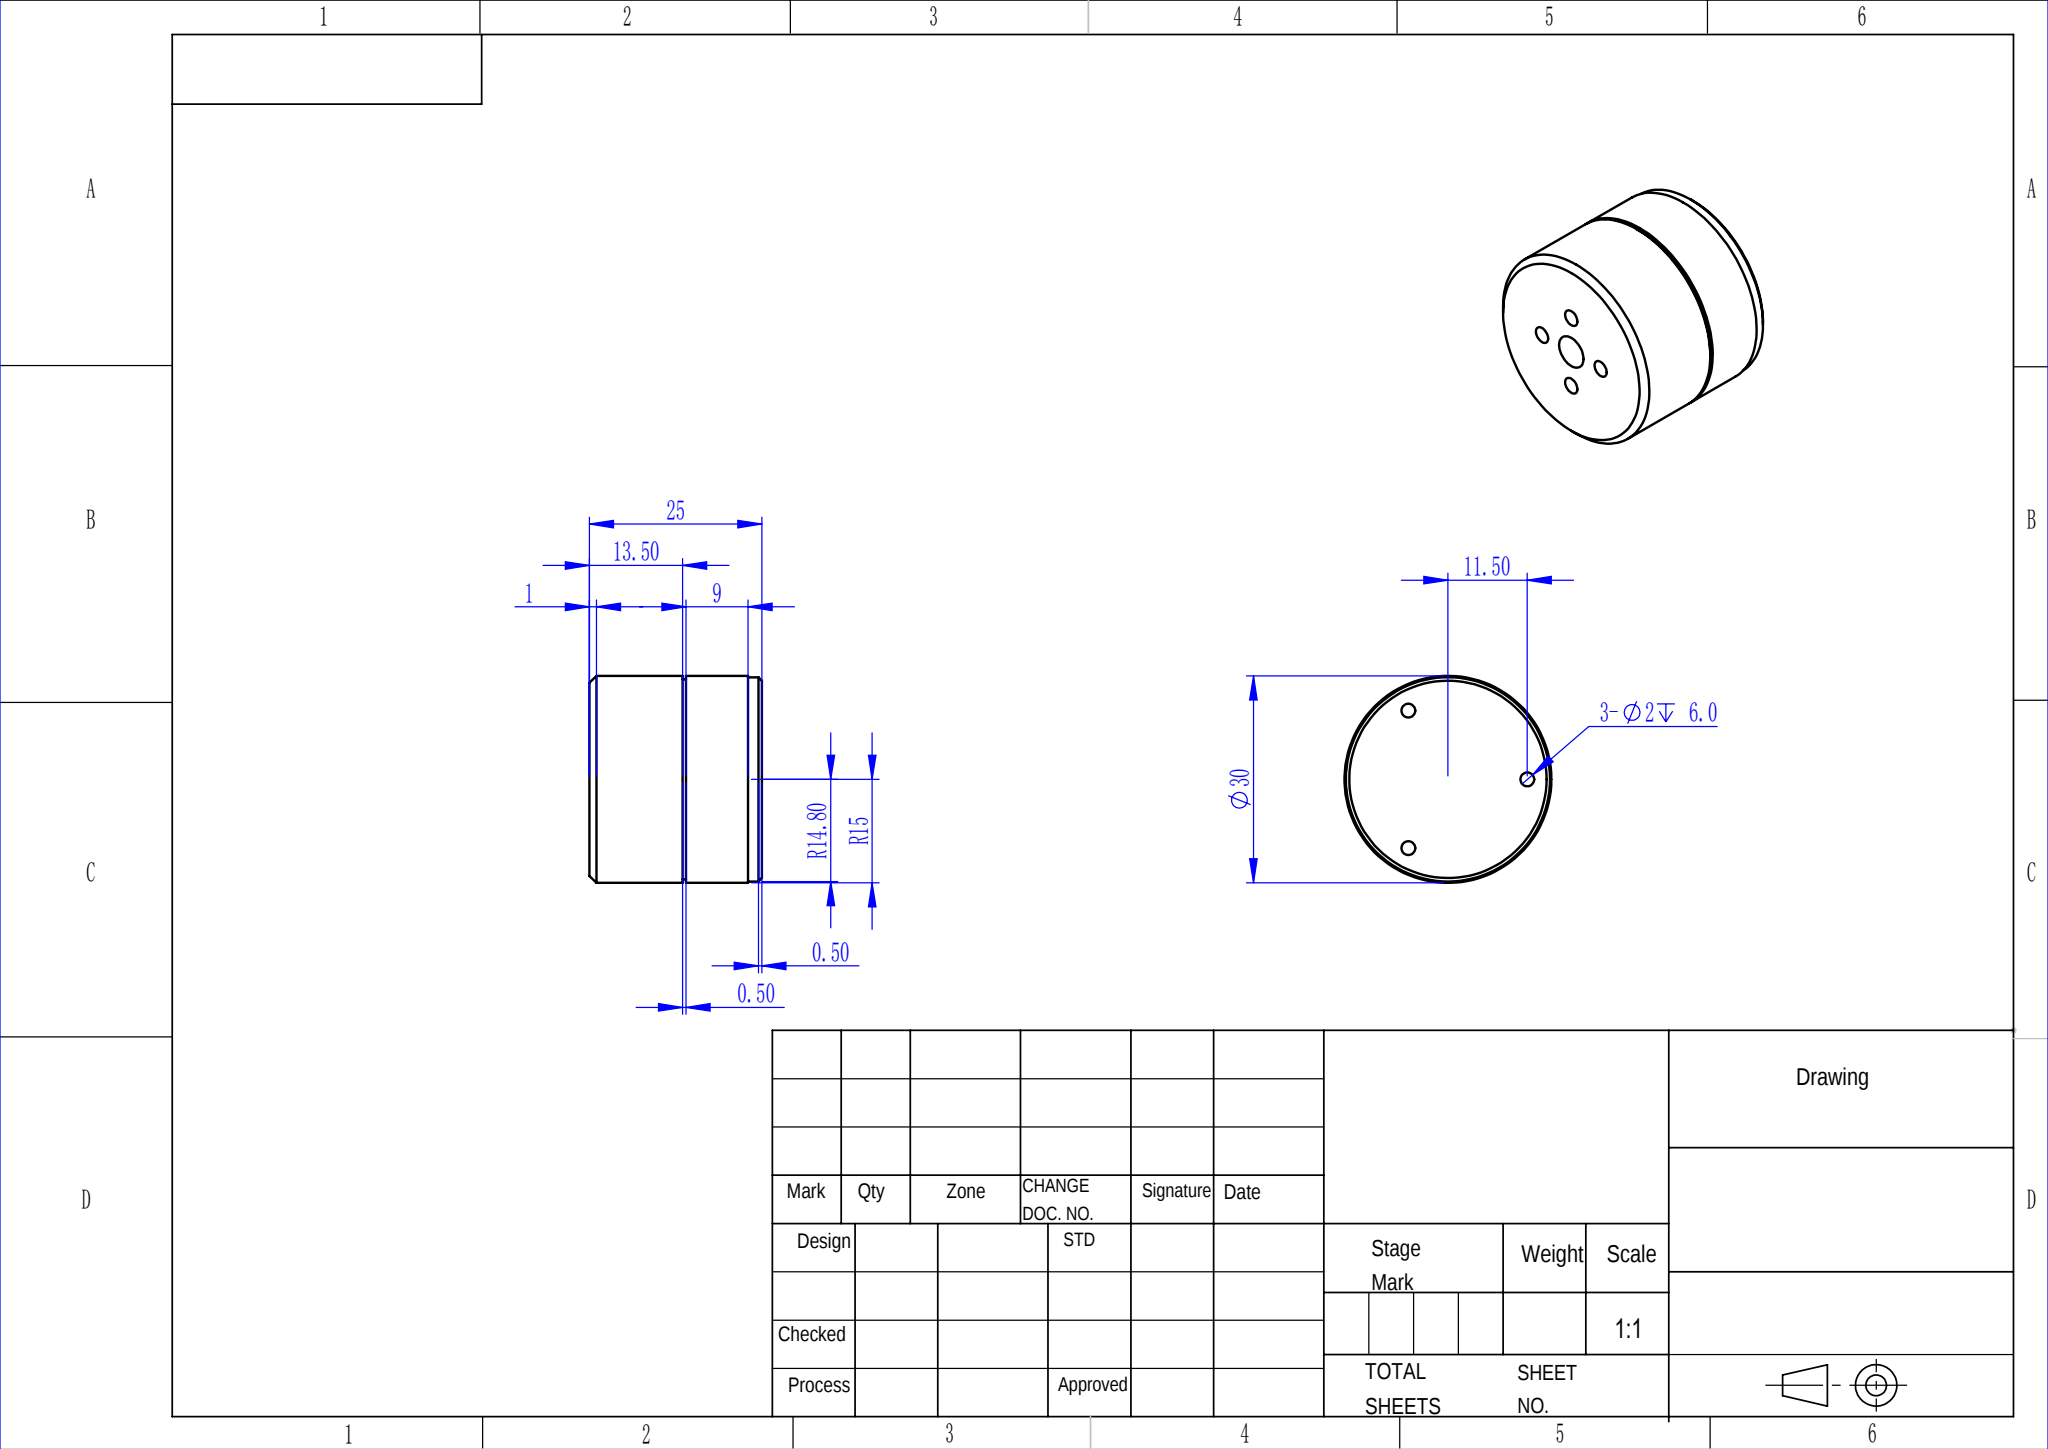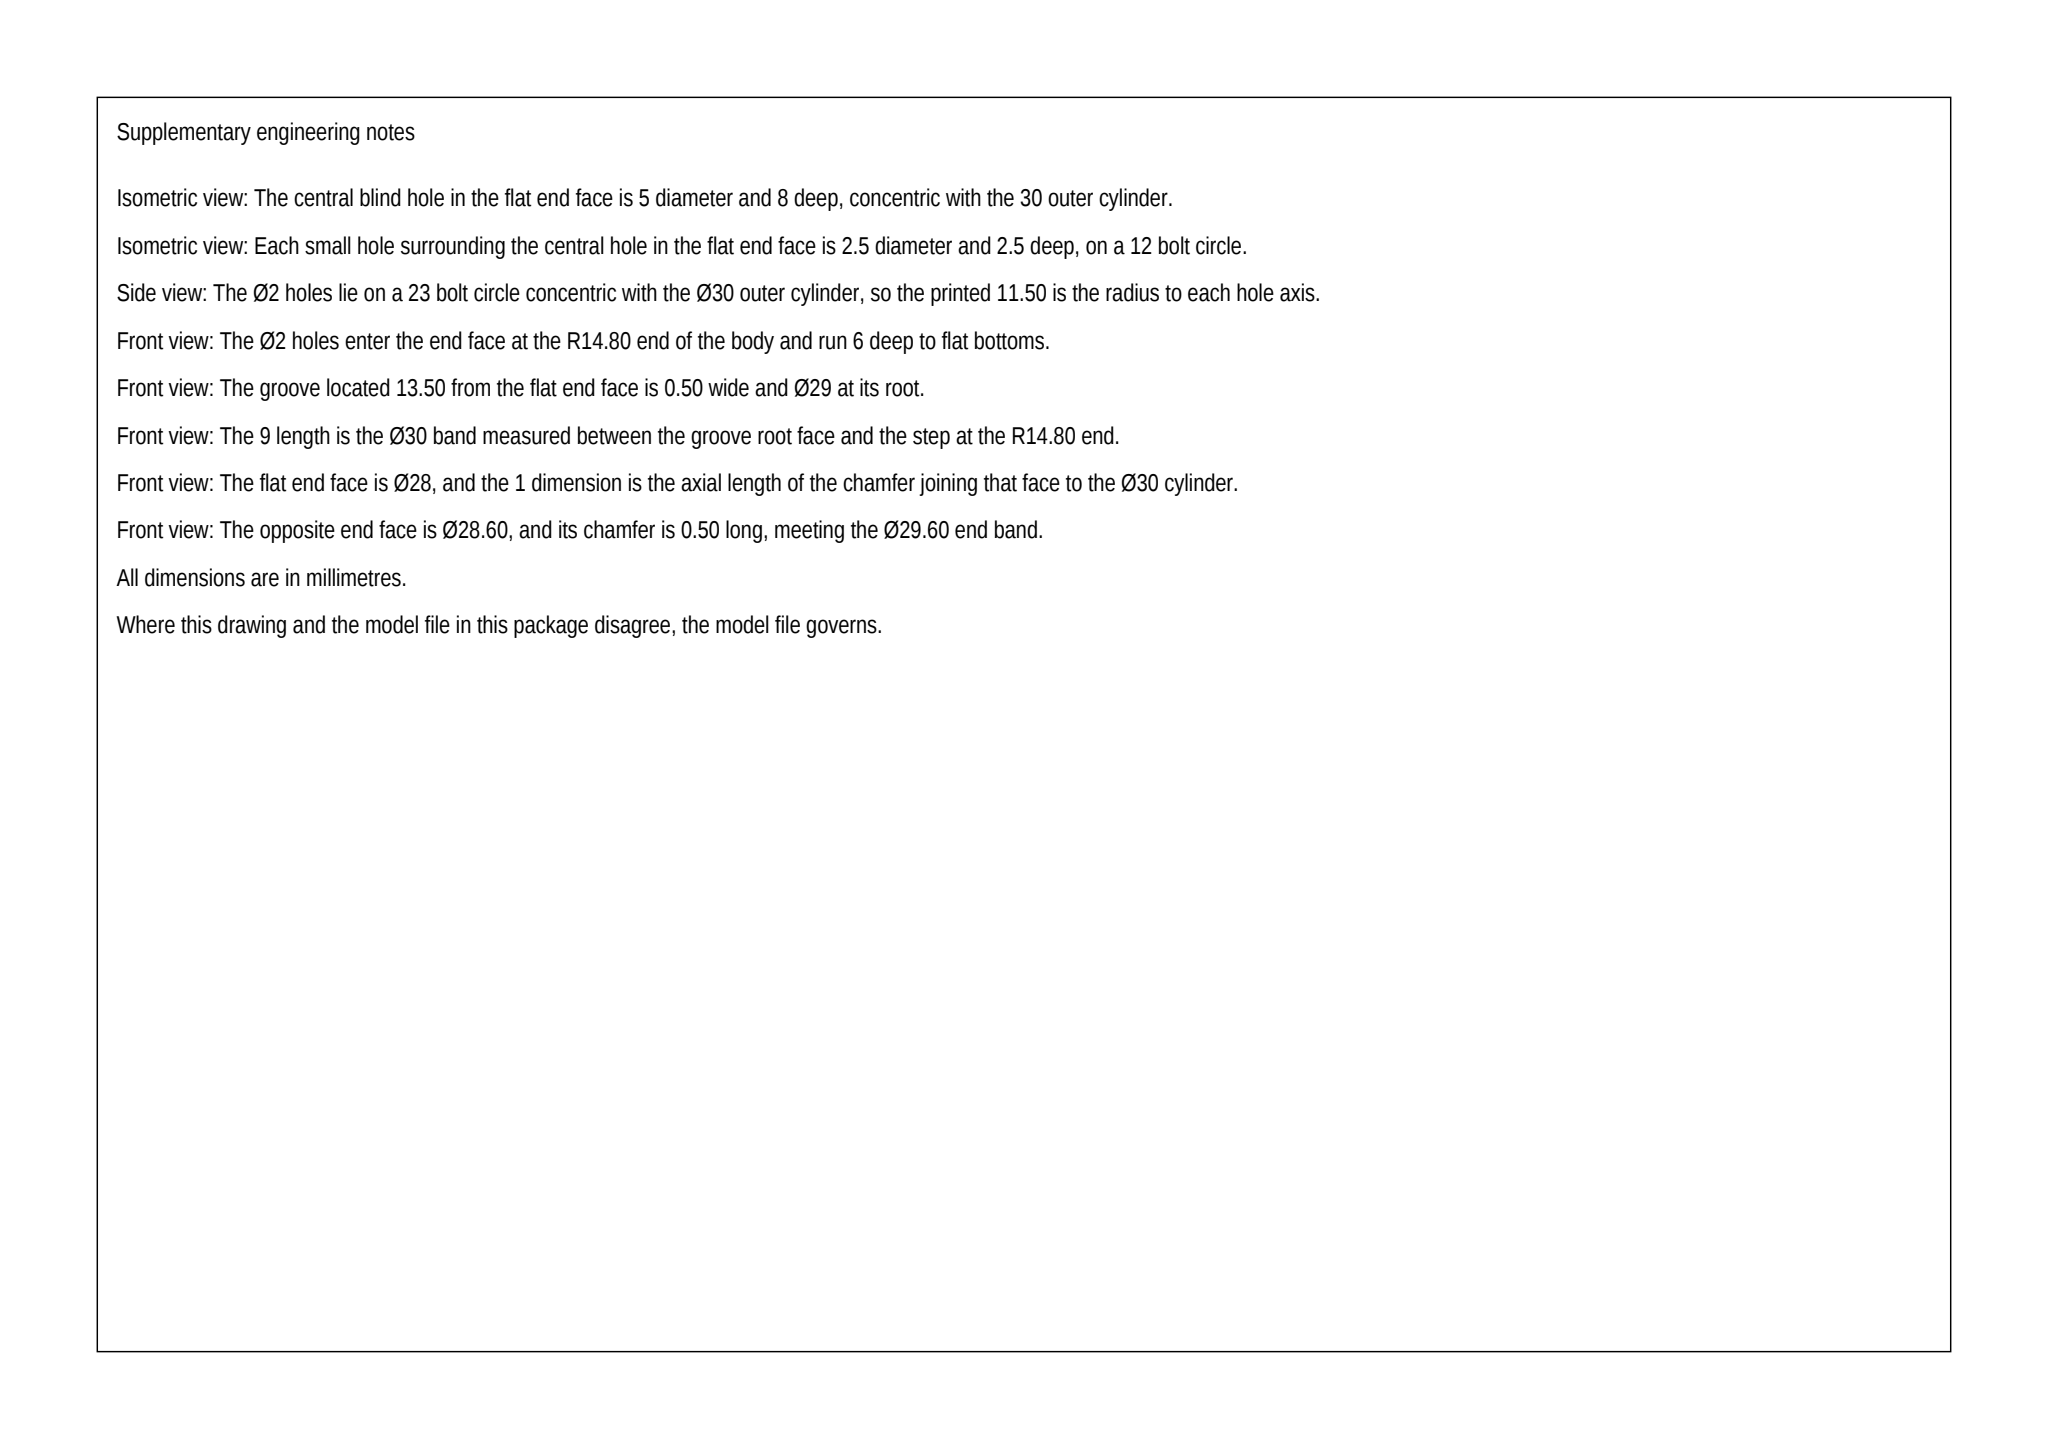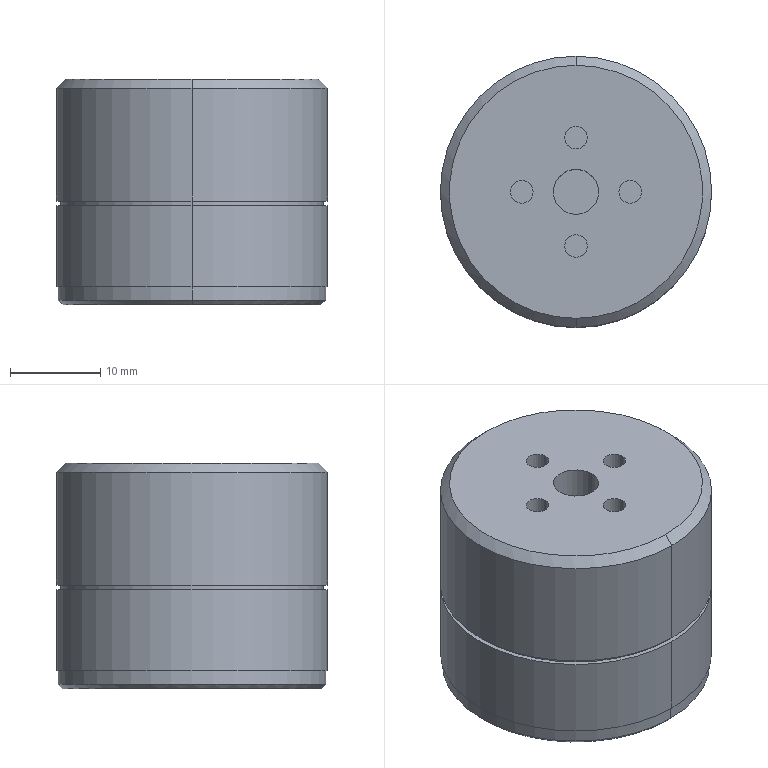Part | SolidWorks | mm | 1 solid | 41 faces | box 30 x 30 x 25 mm | volume 17291 mm3 | cylinder 24 | plane 13 | cone 4 | commonest cylinder face diameters 2.5 x8 2 x6 30 x4 5 x2 29.6 x2 29 x2
Drawing notes:
Ø5 BLIND HOLE DP 8.0, ON PART AXIS (CENTERED ON Ø30 O.D.), ENTERS FROM THE 4-HOLE END FACE | from the solid: cylinder dia 5.0, axis z, pos (15.0,15.0), length 8.0; z-plane at 17.0 (hole bottom) with end face at z=25.0
4X Ø2.5 DP 2.5, EQUALLY SPACED 90° ON Ø12 BOLT CIRCLE CONCENTRIC WITH Ø30 O.D., ENTERS FROM SAME END FACE AS CENTRAL Ø5 HOLE | from the solid: cylinders dia 2.5, axis z, pos (9,15),(15,9),(15,21),(21,15), length 2.5; z-plane 22.5 (4 bottoms) with end face z=25.0; radius 6.0 from center (15,15)
3X Ø2 DP 6.0 EQUALLY SPACED 120° ON Ø23 BOLT CIRCLE (R11.50) CONCENTRIC WITH Ø30 O.D., ENTERS FROM END FACE OPPOSITE THE Ø5/Ø2.5 HOLE FACE | from the solid: cylinders dia 2.0, axis z, pos (5.04,9.25),(15,26.5),(24.96,9.25), length 6.0, all R11.5 from center at 120°; z-plane 6.0 (3 bottoms) with end face z=0
GROOVE ROOT Ø29.0 (R14.50) x 0.50 WIDE, CONCENTRIC WITH Ø30 O.D., AXIALLY LOCATED PER THE 13.50 DIM FROM THE Ø5/Ø2.5 HOLE END FACE | from the solid: cylinders: [29.0,'z',[15.0,15.0],0.5] concentric with [30.0,'z',[15.0,15.0]]; axis_planes z=11.0 and z=11.5
GROOVE SIDE WALLS 90° INCLUDED ANGLE (45° PER SIDE TO PART AXIS), BLENDING Ø30 O.D. TO Ø29.0 ROOT | from the solid: cones[included_angle,ref_dia]: [90.0,30.0] x2 and [90.0,28.6] x2
GROOVE RADIAL DEPTH 0.50 (Ø30 O.D. TO Ø29.0 ROOT); 0.50 AXIAL DIMS ARE THE 45° WALL RUN-OUT | from the solid: cylinders 30.0 and 29.0 on z axis at [15.0,15.0] give (30.0-29.0)/2 = 0.50 radial; cones included_angle 90.0
RELIEF Ø29.6 x 1.50 LONG ADJACENT TO THE GROOVE, CONCENTRIC WITH Ø30 O.D. | from the solid: cylinders: [29.6,'z',[15.0,15.0],1.5]
45° CHAMFER 0.50 AXIAL x 0.50 RADIAL (Ø29.6 TO Ø28.6) AT THE END FACE OF THE Ø29.6 RELIEF; CHAMFER RUNS FROM 9.00 TO 9.50 FROM THE 3X Ø2 HOLE END FACE (I.E. 15.50 TO 16.00 FROM THE Ø5/Ø2.5 HOLE END FACE), CONCENTRIC WITH Ø30 O.D. THIS 0.50 IS SEPARATE FROM THE GROOVE 45° WALL RUN-OUTS OF NOTE 6 | from the solid: cones[included_angle 90.0, ref_dia 28.6] together with cylinders Ø30 x 9.0 and Ø29.6 x 1.5 on z axis (bbox length 25.0; Ø2 holes dp 6.0 enter at z=0, Ø5 dp 8.0 / Ø2.5 dp 2.5 enter at z=25)
build123d program:
from build123d import *

# Parameters (mm, degrees)
SKETCH3_R          = 1
CUT_EXTRUDE1_DEPTH = 6
SKETCH4_R          = 1.25
CUT_EXTRUDE2_DEPTH = 2.5
SKETCH5_R          = 2.5
CUT_EXTRUDE3_DEPTH = 8


with BuildPart() as part:
    # Sketch2 → Revolve1 (revolve)
    with BuildSketch(Plane(origin=(0, 0, 0), x_dir=(0, 0, -1), z_dir=(1, 0, 0))):
        Polygon((0, 0), (0, 14), (1, 15), (13.5, 15), (13.5, 14.5), (14, 14.5), (14, 15), (23, 15), (23, 14.8), (24.5, 14.8), (25, 14.3), (25, 0), align=None)
    revolve(axis=Axis((0, 0, -25), (0, 0, 1)))

    # Sketch3 → Cut-Extrude1 (cut)
    with BuildSketch(Plane(origin=(0, 0, -25), x_dir=(-1, 0, 0), z_dir=(0, 0, -1))):
        with Locations(Location((9.959, -5.75, 0), (0, 0, 90))):
            Circle(SKETCH3_R)
        with Locations(Location((-9.959, -5.75, 0), (0, 0, 90))):
            Circle(SKETCH3_R)
        with Locations(Location((0, 11.5, 0), (0, 0, 90))):
            Circle(SKETCH3_R)
    extrude(amount=-CUT_EXTRUDE1_DEPTH, mode=Mode.SUBTRACT)

    # Sketch4 → Cut-Extrude2 (cut)
    with BuildSketch(Plane.XY):
        with Locations((0, 6)):
            Circle(SKETCH4_R)
        with Locations((6, 0)):
            Circle(SKETCH4_R)
        with Locations((0, -6)):
            Circle(SKETCH4_R)
        with Locations((-6, 0)):
            Circle(SKETCH4_R)
    extrude(amount=-CUT_EXTRUDE2_DEPTH, mode=Mode.SUBTRACT)

    # Sketch5 → Cut-Extrude3 (cut)
    with BuildSketch(Plane.XY):
        Circle(SKETCH5_R)
    extrude(amount=-CUT_EXTRUDE3_DEPTH, mode=Mode.SUBTRACT)


solid = part.part